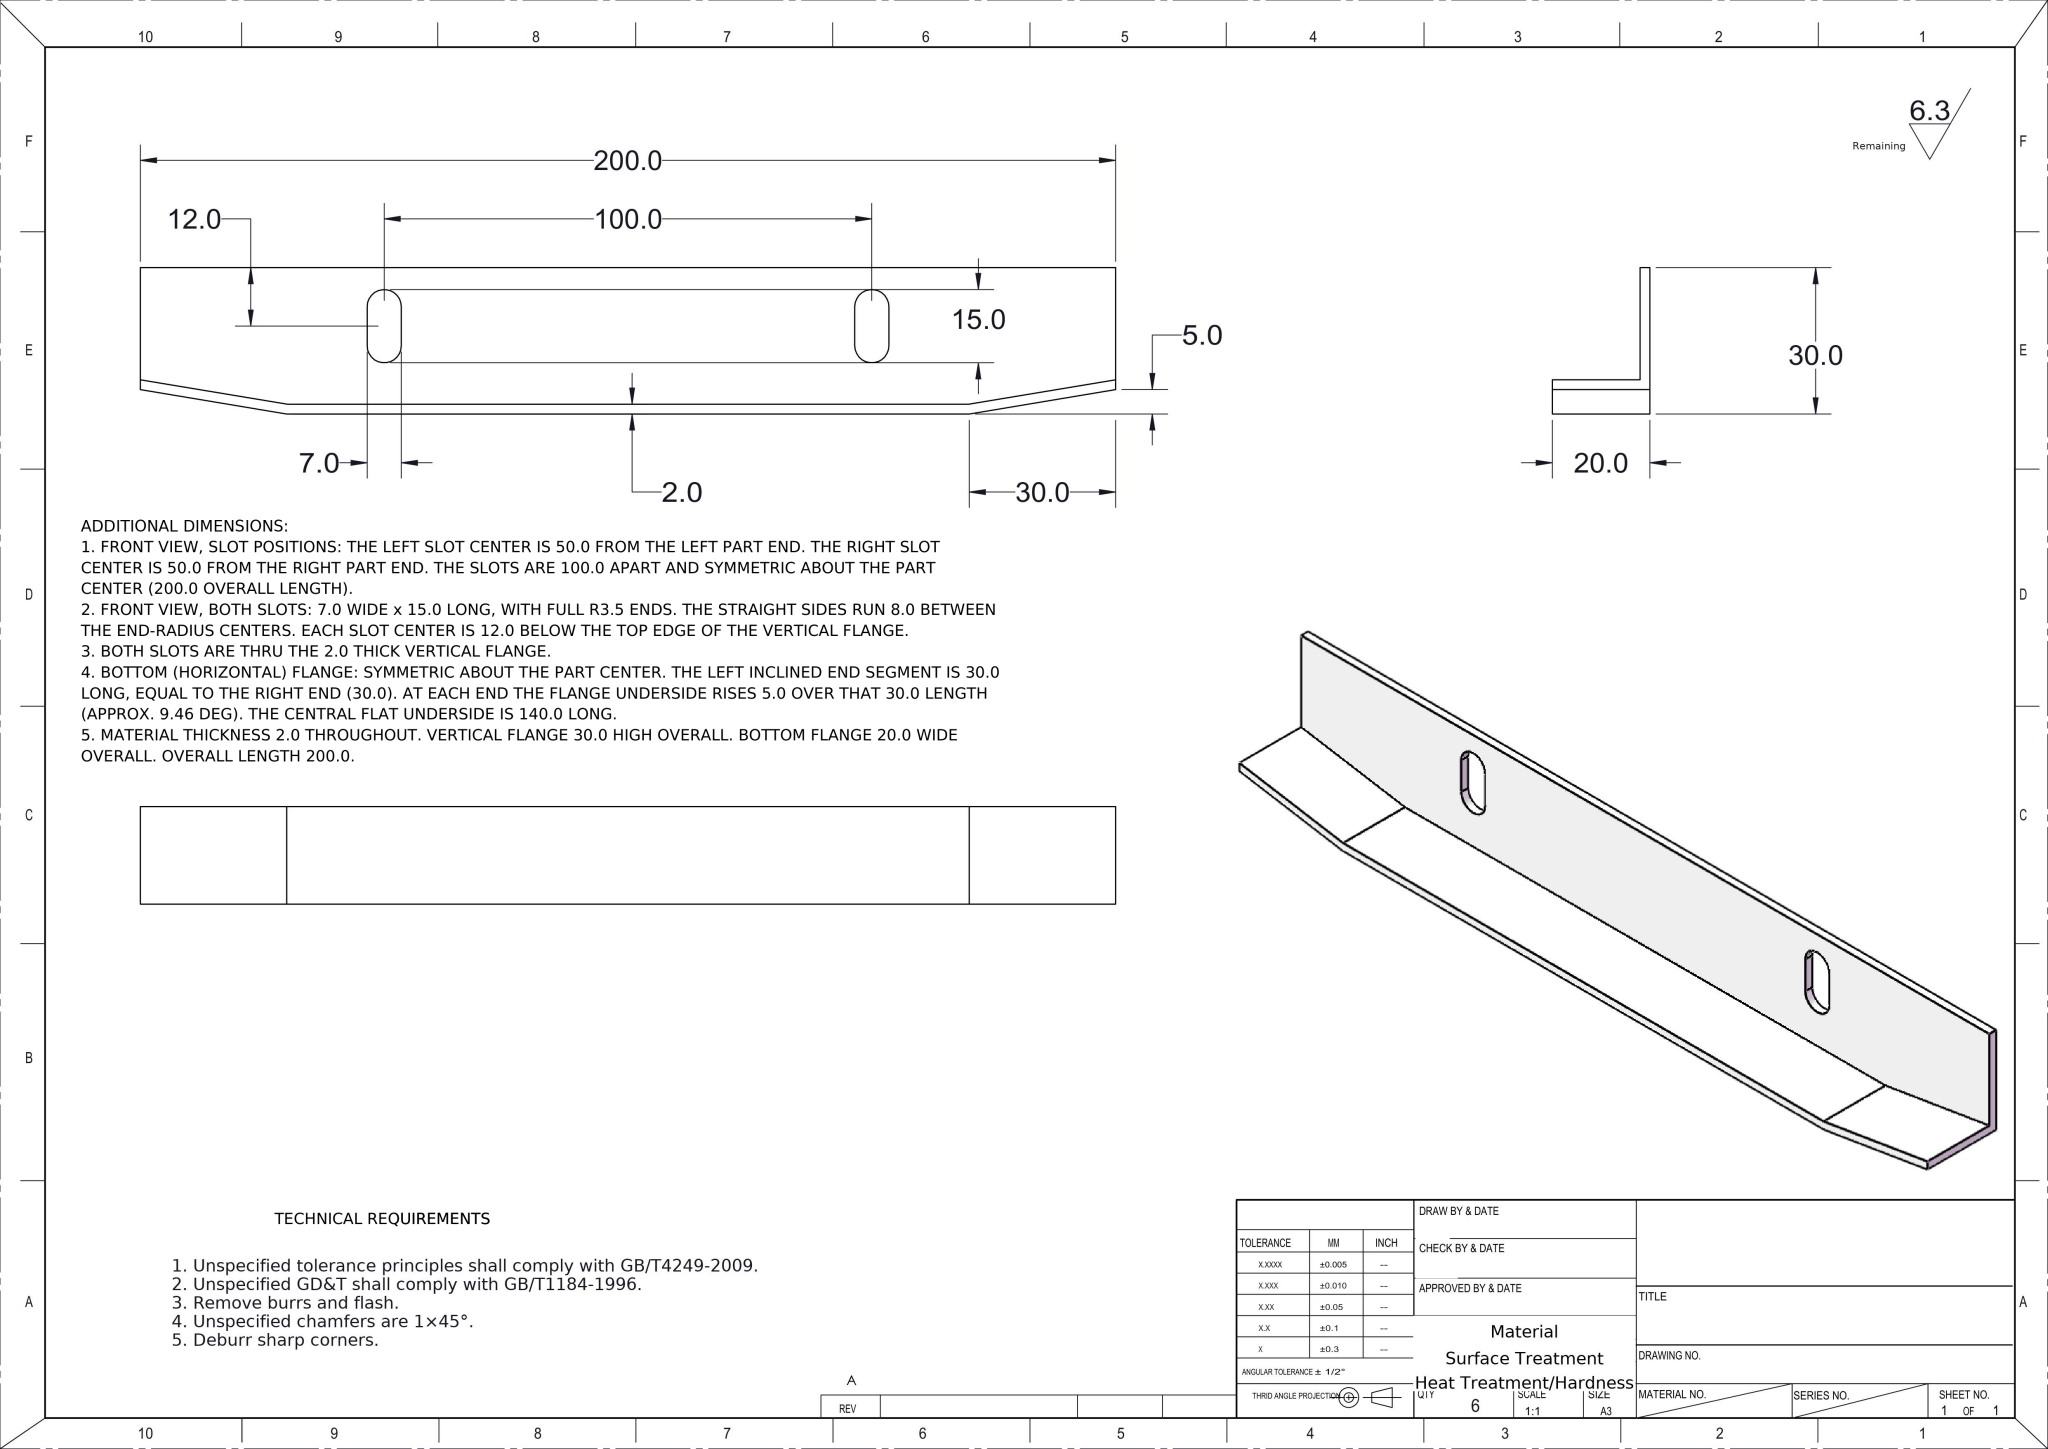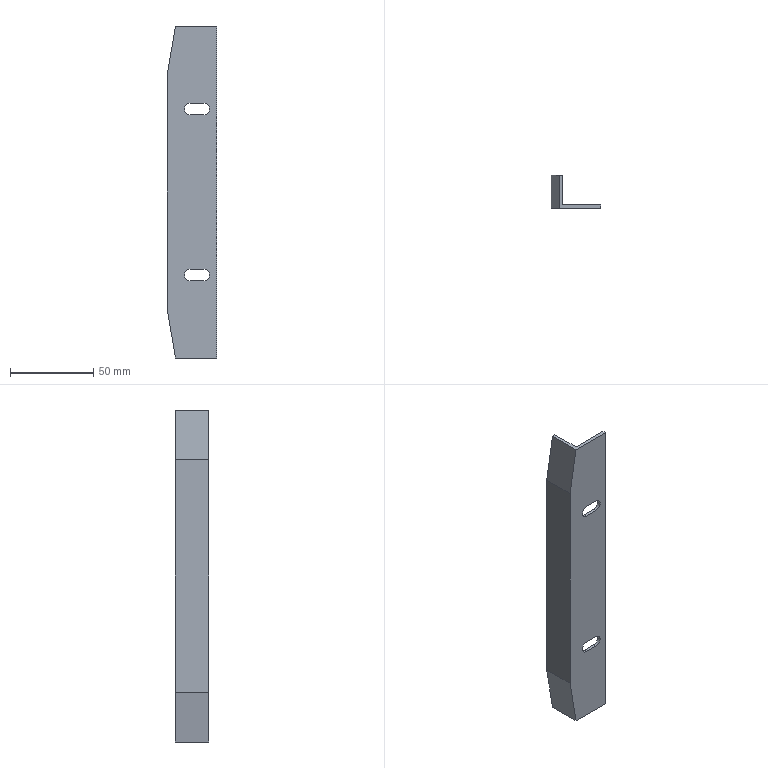Part | NX | mm | Angled Top Mounting Bracket | 1 solid | 20 faces | box 30 x 20 x 200 mm | volume 18552 mm3 | plane 16 | cylinder 4 | commonest cylinder face diameters 7 x4
STEP:
#1=COLOUR_RGB('',1.,1.,1.);
#2=FILL_AREA_STYLE_COLOUR('',#1);
#3=FILL_AREA_STYLE('',(#2));
#4=SURFACE_STYLE_FILL_AREA(#3);
#5=SURFACE_SIDE_STYLE('',(#4));
#6=SURFACE_STYLE_USAGE(.BOTH.,#5);
#7=PRESENTATION_STYLE_ASSIGNMENT((#6));
#8=CARTESIAN_POINT('',(7.028,20.,-100.));
#9=VERTEX_POINT('',#8);
#10=CARTESIAN_POINT('',(2.,20.,-69.834));
#11=VERTEX_POINT('',#10);
#12=CARTESIAN_POINT('',(1.973,20.,-69.671));
#13=DIRECTION('',(-0.1644,0.,0.9864));
#14=VECTOR('',#13,1000.);
#15=LINE('',#12,#14);
#16=EDGE_CURVE('',#9,#11,#15,.T.);
#17=ORIENTED_EDGE('',*,*,#16,.F.);
#18=CARTESIAN_POINT('',(5.,20.,-100.));
#19=VERTEX_POINT('',#18);
#20=CARTESIAN_POINT('',(0.,20.,-100.));
#21=DIRECTION('',(-1.,0.,0.));
#22=VECTOR('',#21,1000.);
#23=LINE('',#20,#22);
#24=EDGE_CURVE('',#9,#19,#23,.T.);
#25=ORIENTED_EDGE('',*,*,#24,.T.);
#26=CARTESIAN_POINT('',(0.,20.,-70.));
#27=VERTEX_POINT('',#26);
#28=CARTESIAN_POINT('',(0.,20.,-70.));
#29=DIRECTION('',(-0.1644,0.,0.9864));
#30=VECTOR('',#29,1000.);
#31=LINE('',#28,#30);
#32=EDGE_CURVE('',#19,#27,#31,.T.);
#33=ORIENTED_EDGE('',*,*,#32,.T.);
#34=CARTESIAN_POINT('',(0.,20.,70.));
#35=VERTEX_POINT('',#34);
#36=CARTESIAN_POINT('',(0.,20.,100.));
#37=DIRECTION('',(0.,0.,-1.));
#38=VECTOR('',#37,1000.);
#39=LINE('',#36,#38);
#40=EDGE_CURVE('',#35,#27,#39,.T.);
#41=ORIENTED_EDGE('',*,*,#40,.F.);
#42=CARTESIAN_POINT('',(5.,20.,100.));
#43=VERTEX_POINT('',#42);
#44=CARTESIAN_POINT('',(0.,20.,70.));
#45=DIRECTION('',(-0.1644,0.,-0.9864));
#46=VECTOR('',#45,1000.);
#47=LINE('',#44,#46);
#48=EDGE_CURVE('',#43,#35,#47,.T.);
#49=ORIENTED_EDGE('',*,*,#48,.F.);
#50=CARTESIAN_POINT('',(7.028,20.,100.));
#51=VERTEX_POINT('',#50);
#52=CARTESIAN_POINT('',(0.,20.,100.));
#53=DIRECTION('',(-1.,0.,0.));
#54=VECTOR('',#53,1000.);
#55=LINE('',#52,#54);
#56=EDGE_CURVE('',#51,#43,#55,.T.);
#57=ORIENTED_EDGE('',*,*,#56,.F.);
#58=CARTESIAN_POINT('',(2.,20.,69.834));
#59=VERTEX_POINT('',#58);
#60=CARTESIAN_POINT('',(1.973,20.,69.671));
#61=DIRECTION('',(-0.1644,0.,-0.9864));
#62=VECTOR('',#61,1000.);
#63=LINE('',#60,#62);
#64=EDGE_CURVE('',#51,#59,#63,.T.);
#65=ORIENTED_EDGE('',*,*,#64,.T.);
#66=CARTESIAN_POINT('',(2.,20.,100.));
#67=DIRECTION('',(0.,0.,-1.));
#68=VECTOR('',#67,1000.);
#69=LINE('',#66,#68);
#70=EDGE_CURVE('',#59,#11,#69,.T.);
#71=ORIENTED_EDGE('',*,*,#70,.T.);
#72=EDGE_LOOP('',(#17,#25,#33,#41,#49,#57,#65,#71));
#73=FACE_OUTER_BOUND('',#72,.T.);
#74=CARTESIAN_POINT('',(0.,20.,100.));
#75=DIRECTION('',(0.,-1.,0.));
#76=DIRECTION('',(0.,0.,-1.));
#77=AXIS2_PLACEMENT_3D('',#74,#75,#76);
#78=PLANE('',#77);
#79=ADVANCED_FACE('',(#73),#78,.F.);
#80=CARTESIAN_POINT('',(7.028,2.,-100.));
#81=VERTEX_POINT('',#80);
#82=CARTESIAN_POINT('',(7.028,0.,-100.));
#83=DIRECTION('',(0.,1.,0.));
#84=VECTOR('',#83,1000.);
#85=LINE('',#82,#84);
#86=EDGE_CURVE('',#81,#9,#85,.T.);
#87=ORIENTED_EDGE('',*,*,#86,.F.);
#88=CARTESIAN_POINT('',(30.,2.,-100.));
#89=VERTEX_POINT('',#88);
#90=CARTESIAN_POINT('',(0.,2.,-100.));
#91=DIRECTION('',(1.,0.,0.));
#92=VECTOR('',#91,1000.);
#93=LINE('',#90,#92);
#94=EDGE_CURVE('',#81,#89,#93,.T.);
#95=ORIENTED_EDGE('',*,*,#94,.T.);
#96=CARTESIAN_POINT('',(30.,0.,-100.));
#97=VERTEX_POINT('',#96);
#98=CARTESIAN_POINT('',(30.,20.,-100.));
#99=DIRECTION('',(-0.,1.,0.));
#100=VECTOR('',#99,1000.);
#101=LINE('',#98,#100);
#102=EDGE_CURVE('',#97,#89,#101,.T.);
#103=ORIENTED_EDGE('',*,*,#102,.F.);
#104=CARTESIAN_POINT('',(5.,0.,-100.));
#105=VERTEX_POINT('',#104);
#106=CARTESIAN_POINT('',(0.,0.,-100.));
#107=DIRECTION('',(1.,0.,0.));
#108=VECTOR('',#107,1000.);
#109=LINE('',#106,#108);
#110=EDGE_CURVE('',#105,#97,#109,.T.);
#111=ORIENTED_EDGE('',*,*,#110,.F.);
#112=CARTESIAN_POINT('',(5.,0.,-100.));
#113=DIRECTION('',(0.,1.,0.));
#114=VECTOR('',#113,1000.);
#115=LINE('',#112,#114);
#116=EDGE_CURVE('',#105,#19,#115,.T.);
#117=ORIENTED_EDGE('',*,*,#116,.T.);
#118=ORIENTED_EDGE('',*,*,#24,.F.);
#119=EDGE_LOOP('',(#87,#95,#103,#111,#117,#118));
#120=FACE_OUTER_BOUND('',#119,.T.);
#121=CARTESIAN_POINT('',(0.,0.,-100.));
#122=DIRECTION('',(0.,0.,-1.));
#123=DIRECTION('',(-1.,0.,0.));
#124=AXIS2_PLACEMENT_3D('',#121,#122,#123);
#125=PLANE('',#124);
#126=ADVANCED_FACE('',(#120),#125,.T.);
#127=CARTESIAN_POINT('',(30.,2.,100.));
#128=VERTEX_POINT('',#127);
#129=CARTESIAN_POINT('',(30.,2.,100.));
#130=DIRECTION('',(0.,0.,-1.));
#131=VECTOR('',#130,1000.);
#132=LINE('',#129,#131);
#133=EDGE_CURVE('',#128,#89,#132,.T.);
#134=ORIENTED_EDGE('',*,*,#133,.F.);
#135=CARTESIAN_POINT('',(30.,0.,100.));
#136=VERTEX_POINT('',#135);
#137=CARTESIAN_POINT('',(30.,20.,100.));
#138=DIRECTION('',(-0.,1.,0.));
#139=VECTOR('',#138,1000.);
#140=LINE('',#137,#139);
#141=EDGE_CURVE('',#136,#128,#140,.T.);
#142=ORIENTED_EDGE('',*,*,#141,.F.);
#143=CARTESIAN_POINT('',(30.,0.,100.));
#144=DIRECTION('',(0.,0.,-1.));
#145=VECTOR('',#144,1000.);
#146=LINE('',#143,#145);
#147=EDGE_CURVE('',#136,#97,#146,.T.);
#148=ORIENTED_EDGE('',*,*,#147,.T.);
#149=ORIENTED_EDGE('',*,*,#102,.T.);
#150=EDGE_LOOP('',(#134,#142,#148,#149));
#151=FACE_OUTER_BOUND('',#150,.T.);
#152=CARTESIAN_POINT('',(30.,20.,100.));
#153=DIRECTION('',(-1.,-0.,0.));
#154=DIRECTION('',(0.,-1.,0.));
#155=AXIS2_PLACEMENT_3D('',#152,#153,#154);
#156=PLANE('',#155);
#157=ADVANCED_FACE('',(#151),#156,.F.);
#158=CARTESIAN_POINT('',(0.,0.,-70.));
#159=VERTEX_POINT('',#158);
#160=CARTESIAN_POINT('',(0.,0.,-70.));
#161=DIRECTION('',(0.,1.,0.));
#162=VECTOR('',#161,1000.);
#163=LINE('',#160,#162);
#164=EDGE_CURVE('',#159,#27,#163,.T.);
#165=ORIENTED_EDGE('',*,*,#164,.F.);
#166=CARTESIAN_POINT('',(0.,0.,70.));
#167=VERTEX_POINT('',#166);
#168=CARTESIAN_POINT('',(0.,0.,100.));
#169=DIRECTION('',(0.,0.,-1.));
#170=VECTOR('',#169,1000.);
#171=LINE('',#168,#170);
#172=EDGE_CURVE('',#167,#159,#171,.T.);
#173=ORIENTED_EDGE('',*,*,#172,.F.);
#174=CARTESIAN_POINT('',(0.,0.,70.));
#175=DIRECTION('',(0.,1.,0.));
#176=VECTOR('',#175,1000.);
#177=LINE('',#174,#176);
#178=EDGE_CURVE('',#167,#35,#177,.T.);
#179=ORIENTED_EDGE('',*,*,#178,.T.);
#180=ORIENTED_EDGE('',*,*,#40,.T.);
#181=EDGE_LOOP('',(#165,#173,#179,#180));
#182=FACE_OUTER_BOUND('',#181,.T.);
#183=CARTESIAN_POINT('',(0.,20.,100.));
#184=DIRECTION('',(1.,0.,0.));
#185=DIRECTION('',(0.,0.,-1.));
#186=AXIS2_PLACEMENT_3D('',#183,#184,#185);
#187=PLANE('',#186);
#188=ADVANCED_FACE('',(#182),#187,.F.);
#189=CARTESIAN_POINT('',(22.,0.,-46.5));
#190=VERTEX_POINT('',#189);
#191=CARTESIAN_POINT('',(14.,0.,-46.5));
#192=VERTEX_POINT('',#191);
#193=CARTESIAN_POINT('',(22.,0.,-46.5));
#194=DIRECTION('',(-1.,0.,0.));
#195=VECTOR('',#194,1000.);
#196=LINE('',#193,#195);
#197=EDGE_CURVE('',#190,#192,#196,.T.);
#198=ORIENTED_EDGE('',*,*,#197,.F.);
#199=CARTESIAN_POINT('',(22.,0.,-53.5));
#200=VERTEX_POINT('',#199);
#201=CARTESIAN_POINT('',(22.,0.,-50.));
#202=DIRECTION('',(0.,-1.,0.));
#203=DIRECTION('',(0.,0.,1.));
#204=AXIS2_PLACEMENT_3D('',#201,#202,#203);
#205=CIRCLE('',#204,3.5);
#206=EDGE_CURVE('',#200,#190,#205,.T.);
#207=ORIENTED_EDGE('',*,*,#206,.F.);
#208=CARTESIAN_POINT('',(14.,0.,-53.5));
#209=VERTEX_POINT('',#208);
#210=CARTESIAN_POINT('',(22.,0.,-53.5));
#211=DIRECTION('',(1.,0.,0.));
#212=VECTOR('',#211,1000.);
#213=LINE('',#210,#212);
#214=EDGE_CURVE('',#209,#200,#213,.T.);
#215=ORIENTED_EDGE('',*,*,#214,.F.);
#216=CARTESIAN_POINT('',(14.,0.,-50.));
#217=DIRECTION('',(0.,-1.,0.));
#218=DIRECTION('',(0.,0.,1.));
#219=AXIS2_PLACEMENT_3D('',#216,#217,#218);
#220=CIRCLE('',#219,3.5);
#221=EDGE_CURVE('',#192,#209,#220,.T.);
#222=ORIENTED_EDGE('',*,*,#221,.F.);
#223=EDGE_LOOP('',(#198,#207,#215,#222));
#224=FACE_BOUND('',#223,.T.);
#225=CARTESIAN_POINT('',(22.,0.,53.5));
#226=VERTEX_POINT('',#225);
#227=CARTESIAN_POINT('',(14.,0.,53.5));
#228=VERTEX_POINT('',#227);
#229=CARTESIAN_POINT('',(22.,0.,53.5));
#230=DIRECTION('',(-1.,0.,0.));
#231=VECTOR('',#230,1000.);
#232=LINE('',#229,#231);
#233=EDGE_CURVE('',#226,#228,#232,.T.);
#234=ORIENTED_EDGE('',*,*,#233,.F.);
#235=CARTESIAN_POINT('',(22.,0.,46.5));
#236=VERTEX_POINT('',#235);
#237=CARTESIAN_POINT('',(22.,0.,50.));
#238=DIRECTION('',(0.,-1.,0.));
#239=DIRECTION('',(0.,0.,-1.));
#240=AXIS2_PLACEMENT_3D('',#237,#238,#239);
#241=CIRCLE('',#240,3.5);
#242=EDGE_CURVE('',#236,#226,#241,.T.);
#243=ORIENTED_EDGE('',*,*,#242,.F.);
#244=CARTESIAN_POINT('',(14.,0.,46.5));
#245=VERTEX_POINT('',#244);
#246=CARTESIAN_POINT('',(22.,0.,46.5));
#247=DIRECTION('',(1.,0.,0.));
#248=VECTOR('',#247,1000.);
#249=LINE('',#246,#248);
#250=EDGE_CURVE('',#245,#236,#249,.T.);
#251=ORIENTED_EDGE('',*,*,#250,.F.);
#252=CARTESIAN_POINT('',(14.,0.,50.));
#253=DIRECTION('',(0.,-1.,0.));
#254=DIRECTION('',(0.,0.,-1.));
#255=AXIS2_PLACEMENT_3D('',#252,#253,#254);
#256=CIRCLE('',#255,3.5);
#257=EDGE_CURVE('',#228,#245,#256,.T.);
#258=ORIENTED_EDGE('',*,*,#257,.F.);
#259=EDGE_LOOP('',(#234,#243,#251,#258));
#260=FACE_BOUND('',#259,.T.);
#261=CARTESIAN_POINT('',(0.,0.,-70.));
#262=DIRECTION('',(-0.1644,0.,0.9864));
#263=VECTOR('',#262,1000.);
#264=LINE('',#261,#263);
#265=EDGE_CURVE('',#105,#159,#264,.T.);
#266=ORIENTED_EDGE('',*,*,#265,.F.);
#267=ORIENTED_EDGE('',*,*,#110,.T.);
#268=ORIENTED_EDGE('',*,*,#147,.F.);
#269=CARTESIAN_POINT('',(5.,0.,100.));
#270=VERTEX_POINT('',#269);
#271=CARTESIAN_POINT('',(0.,0.,100.));
#272=DIRECTION('',(1.,0.,0.));
#273=VECTOR('',#272,1000.);
#274=LINE('',#271,#273);
#275=EDGE_CURVE('',#270,#136,#274,.T.);
#276=ORIENTED_EDGE('',*,*,#275,.F.);
#277=CARTESIAN_POINT('',(0.,0.,70.));
#278=DIRECTION('',(-0.1644,0.,-0.9864));
#279=VECTOR('',#278,1000.);
#280=LINE('',#277,#279);
#281=EDGE_CURVE('',#270,#167,#280,.T.);
#282=ORIENTED_EDGE('',*,*,#281,.T.);
#283=ORIENTED_EDGE('',*,*,#172,.T.);
#284=EDGE_LOOP('',(#266,#267,#268,#276,#282,#283));
#285=FACE_OUTER_BOUND('',#284,.T.);
#286=CARTESIAN_POINT('',(0.,0.,100.));
#287=DIRECTION('',(0.,1.,0.));
#288=DIRECTION('',(0.,0.,1.));
#289=AXIS2_PLACEMENT_3D('',#286,#287,#288);
#290=PLANE('',#289);
#291=ADVANCED_FACE('',(#224,#260,#285),#290,.F.);
#292=CARTESIAN_POINT('',(7.028,2.,100.));
#293=VERTEX_POINT('',#292);
#294=CARTESIAN_POINT('',(0.,2.,100.));
#295=DIRECTION('',(1.,0.,0.));
#296=VECTOR('',#295,1000.);
#297=LINE('',#294,#296);
#298=EDGE_CURVE('',#293,#128,#297,.T.);
#299=ORIENTED_EDGE('',*,*,#298,.F.);
#300=CARTESIAN_POINT('',(7.028,0.,100.));
#301=DIRECTION('',(0.,1.,0.));
#302=VECTOR('',#301,1000.);
#303=LINE('',#300,#302);
#304=EDGE_CURVE('',#293,#51,#303,.T.);
#305=ORIENTED_EDGE('',*,*,#304,.T.);
#306=ORIENTED_EDGE('',*,*,#56,.T.);
#307=CARTESIAN_POINT('',(5.,0.,100.));
#308=DIRECTION('',(0.,1.,0.));
#309=VECTOR('',#308,1000.);
#310=LINE('',#307,#309);
#311=EDGE_CURVE('',#270,#43,#310,.T.);
#312=ORIENTED_EDGE('',*,*,#311,.F.);
#313=ORIENTED_EDGE('',*,*,#275,.T.);
#314=ORIENTED_EDGE('',*,*,#141,.T.);
#315=EDGE_LOOP('',(#299,#305,#306,#312,#313,#314));
#316=FACE_OUTER_BOUND('',#315,.T.);
#317=CARTESIAN_POINT('',(0.,0.,100.));
#318=DIRECTION('',(0.,0.,-1.));
#319=DIRECTION('',(-1.,0.,0.));
#320=AXIS2_PLACEMENT_3D('',#317,#318,#319);
#321=PLANE('',#320);
#322=ADVANCED_FACE('',(#316),#321,.F.);
#323=ORIENTED_EDGE('',*,*,#48,.T.);
#324=ORIENTED_EDGE('',*,*,#178,.F.);
#325=ORIENTED_EDGE('',*,*,#281,.F.);
#326=ORIENTED_EDGE('',*,*,#311,.T.);
#327=EDGE_LOOP('',(#323,#324,#325,#326));
#328=FACE_OUTER_BOUND('',#327,.T.);
#329=CARTESIAN_POINT('',(0.,0.,70.));
#330=DIRECTION('',(0.9864,0.,-0.1644));
#331=DIRECTION('',(-0.1644,0.,-0.9864));
#332=AXIS2_PLACEMENT_3D('',#329,#330,#331);
#333=PLANE('',#332);
#334=ADVANCED_FACE('',(#328),#333,.F.);
#335=ORIENTED_EDGE('',*,*,#32,.F.);
#336=ORIENTED_EDGE('',*,*,#116,.F.);
#337=ORIENTED_EDGE('',*,*,#265,.T.);
#338=ORIENTED_EDGE('',*,*,#164,.T.);
#339=EDGE_LOOP('',(#335,#336,#337,#338));
#340=FACE_OUTER_BOUND('',#339,.T.);
#341=CARTESIAN_POINT('',(0.,0.,-70.));
#342=DIRECTION('',(-0.9864,0.,-0.1644));
#343=DIRECTION('',(-0.1644,0.,0.9864));
#344=AXIS2_PLACEMENT_3D('',#341,#342,#343);
#345=PLANE('',#344);
#346=ADVANCED_FACE('',(#340),#345,.T.);
#347=CARTESIAN_POINT('',(2.,2.,-69.834));
#348=VERTEX_POINT('',#347);
#349=CARTESIAN_POINT('',(2.,20.,-69.834));
#350=DIRECTION('',(0.,1.,0.));
#351=VECTOR('',#350,1000.);
#352=LINE('',#349,#351);
#353=EDGE_CURVE('',#348,#11,#352,.T.);
#354=ORIENTED_EDGE('',*,*,#353,.T.);
#355=ORIENTED_EDGE('',*,*,#70,.F.);
#356=CARTESIAN_POINT('',(2.,2.,69.834));
#357=VERTEX_POINT('',#356);
#358=CARTESIAN_POINT('',(2.,20.,69.834));
#359=DIRECTION('',(0.,1.,0.));
#360=VECTOR('',#359,1000.);
#361=LINE('',#358,#360);
#362=EDGE_CURVE('',#357,#59,#361,.T.);
#363=ORIENTED_EDGE('',*,*,#362,.F.);
#364=CARTESIAN_POINT('',(2.,2.,100.));
#365=DIRECTION('',(0.,0.,-1.));
#366=VECTOR('',#365,1000.);
#367=LINE('',#364,#366);
#368=EDGE_CURVE('',#357,#348,#367,.T.);
#369=ORIENTED_EDGE('',*,*,#368,.T.);
#370=EDGE_LOOP('',(#354,#355,#363,#369));
#371=FACE_OUTER_BOUND('',#370,.T.);
#372=CARTESIAN_POINT('',(2.,20.,100.));
#373=DIRECTION('',(1.,0.,0.));
#374=DIRECTION('',(0.,0.,-1.));
#375=AXIS2_PLACEMENT_3D('',#372,#373,#374);
#376=PLANE('',#375);
#377=ADVANCED_FACE('',(#371),#376,.T.);
#378=CARTESIAN_POINT('',(22.,2.,-53.5));
#379=VERTEX_POINT('',#378);
#380=CARTESIAN_POINT('',(22.,2.,-46.5));
#381=VERTEX_POINT('',#380);
#382=CARTESIAN_POINT('',(22.,2.,-50.));
#383=DIRECTION('',(0.,-1.,0.));
#384=DIRECTION('',(0.,0.,1.));
#385=AXIS2_PLACEMENT_3D('',#382,#383,#384);
#386=CIRCLE('',#385,3.5);
#387=EDGE_CURVE('',#379,#381,#386,.T.);
#388=ORIENTED_EDGE('',*,*,#387,.T.);
#389=CARTESIAN_POINT('',(14.,2.,-46.5));
#390=VERTEX_POINT('',#389);
#391=CARTESIAN_POINT('',(22.,2.,-46.5));
#392=DIRECTION('',(-1.,0.,0.));
#393=VECTOR('',#392,1000.);
#394=LINE('',#391,#393);
#395=EDGE_CURVE('',#381,#390,#394,.T.);
#396=ORIENTED_EDGE('',*,*,#395,.T.);
#397=CARTESIAN_POINT('',(14.,2.,-53.5));
#398=VERTEX_POINT('',#397);
#399=CARTESIAN_POINT('',(14.,2.,-50.));
#400=DIRECTION('',(0.,-1.,0.));
#401=DIRECTION('',(0.,0.,1.));
#402=AXIS2_PLACEMENT_3D('',#399,#400,#401);
#403=CIRCLE('',#402,3.5);
#404=EDGE_CURVE('',#390,#398,#403,.T.);
#405=ORIENTED_EDGE('',*,*,#404,.T.);
#406=CARTESIAN_POINT('',(22.,2.,-53.5));
#407=DIRECTION('',(1.,0.,0.));
#408=VECTOR('',#407,1000.);
#409=LINE('',#406,#408);
#410=EDGE_CURVE('',#398,#379,#409,.T.);
#411=ORIENTED_EDGE('',*,*,#410,.T.);
#412=EDGE_LOOP('',(#388,#396,#405,#411));
#413=FACE_BOUND('',#412,.T.);
#414=CARTESIAN_POINT('',(22.,2.,46.5));
#415=VERTEX_POINT('',#414);
#416=CARTESIAN_POINT('',(22.,2.,53.5));
#417=VERTEX_POINT('',#416);
#418=CARTESIAN_POINT('',(22.,2.,50.));
#419=DIRECTION('',(0.,-1.,0.));
#420=DIRECTION('',(-0.,0.,1.));
#421=AXIS2_PLACEMENT_3D('',#418,#419,#420);
#422=CIRCLE('',#421,3.5);
#423=EDGE_CURVE('',#415,#417,#422,.T.);
#424=ORIENTED_EDGE('',*,*,#423,.T.);
#425=CARTESIAN_POINT('',(14.,2.,53.5));
#426=VERTEX_POINT('',#425);
#427=CARTESIAN_POINT('',(22.,2.,53.5));
#428=DIRECTION('',(-1.,0.,0.));
#429=VECTOR('',#428,1000.);
#430=LINE('',#427,#429);
#431=EDGE_CURVE('',#417,#426,#430,.T.);
#432=ORIENTED_EDGE('',*,*,#431,.T.);
#433=CARTESIAN_POINT('',(14.,2.,46.5));
#434=VERTEX_POINT('',#433);
#435=CARTESIAN_POINT('',(14.,2.,50.));
#436=DIRECTION('',(0.,-1.,0.));
#437=DIRECTION('',(0.,0.,1.));
#438=AXIS2_PLACEMENT_3D('',#435,#436,#437);
#439=CIRCLE('',#438,3.5);
#440=EDGE_CURVE('',#426,#434,#439,.T.);
#441=ORIENTED_EDGE('',*,*,#440,.T.);
#442=CARTESIAN_POINT('',(22.,2.,46.5));
#443=DIRECTION('',(1.,0.,0.));
#444=VECTOR('',#443,1000.);
#445=LINE('',#442,#444);
#446=EDGE_CURVE('',#434,#415,#445,.T.);
#447=ORIENTED_EDGE('',*,*,#446,.T.);
#448=EDGE_LOOP('',(#424,#432,#441,#447));
#449=FACE_BOUND('',#448,.T.);
#450=CARTESIAN_POINT('',(-25.595,2.,95.734));
#451=DIRECTION('',(-0.1644,0.,0.9864));
#452=VECTOR('',#451,1000.);
#453=LINE('',#450,#452);
#454=EDGE_CURVE('',#81,#348,#453,.T.);
#455=ORIENTED_EDGE('',*,*,#454,.T.);
#456=ORIENTED_EDGE('',*,*,#368,.F.);
#457=CARTESIAN_POINT('',(6.838,2.,98.86));
#458=DIRECTION('',(-0.1644,0.,-0.9864));
#459=VECTOR('',#458,1000.);
#460=LINE('',#457,#459);
#461=EDGE_CURVE('',#293,#357,#460,.T.);
#462=ORIENTED_EDGE('',*,*,#461,.F.);
#463=ORIENTED_EDGE('',*,*,#298,.T.);
#464=ORIENTED_EDGE('',*,*,#133,.T.);
#465=ORIENTED_EDGE('',*,*,#94,.F.);
#466=EDGE_LOOP('',(#455,#456,#462,#463,#464,#465));
#467=FACE_OUTER_BOUND('',#466,.T.);
#468=CARTESIAN_POINT('',(0.,2.,100.));
#469=DIRECTION('',(0.,1.,0.));
#470=DIRECTION('',(0.,0.,1.));
#471=AXIS2_PLACEMENT_3D('',#468,#469,#470);
#472=PLANE('',#471);
#473=ADVANCED_FACE('',(#413,#449,#467),#472,.T.);
#474=ORIENTED_EDGE('',*,*,#64,.F.);
#475=ORIENTED_EDGE('',*,*,#304,.F.);
#476=ORIENTED_EDGE('',*,*,#461,.T.);
#477=ORIENTED_EDGE('',*,*,#362,.T.);
#478=EDGE_LOOP('',(#474,#475,#476,#477));
#479=FACE_OUTER_BOUND('',#478,.T.);
#480=CARTESIAN_POINT('',(1.973,0.,69.671));
#481=DIRECTION('',(0.9864,0.,-0.1644));
#482=DIRECTION('',(-0.1644,0.,-0.9864));
#483=AXIS2_PLACEMENT_3D('',#480,#481,#482);
#484=PLANE('',#483);
#485=ADVANCED_FACE('',(#479),#484,.T.);
#486=ORIENTED_EDGE('',*,*,#16,.T.);
#487=ORIENTED_EDGE('',*,*,#353,.F.);
#488=ORIENTED_EDGE('',*,*,#454,.F.);
#489=ORIENTED_EDGE('',*,*,#86,.T.);
#490=EDGE_LOOP('',(#486,#487,#488,#489));
#491=FACE_OUTER_BOUND('',#490,.T.);
#492=CARTESIAN_POINT('',(1.973,0.,-69.671));
#493=DIRECTION('',(-0.9864,0.,-0.1644));
#494=DIRECTION('',(-0.1644,0.,0.9864));
#495=AXIS2_PLACEMENT_3D('',#492,#493,#494);
#496=PLANE('',#495);
#497=ADVANCED_FACE('',(#491),#496,.F.);
#498=CARTESIAN_POINT('',(22.,20.001,46.5));
#499=DIRECTION('',(0.,-1.,0.));
#500=VECTOR('',#499,1000.);
#501=LINE('',#498,#500);
#502=EDGE_CURVE('',#415,#236,#501,.T.);
#503=ORIENTED_EDGE('',*,*,#502,.T.);
#504=ORIENTED_EDGE('',*,*,#242,.T.);
#505=CARTESIAN_POINT('',(22.,20.001,53.5));
#506=DIRECTION('',(0.,-1.,0.));
#507=VECTOR('',#506,1000.);
#508=LINE('',#505,#507);
#509=EDGE_CURVE('',#417,#226,#508,.T.);
#510=ORIENTED_EDGE('',*,*,#509,.F.);
#511=ORIENTED_EDGE('',*,*,#423,.F.);
#512=EDGE_LOOP('',(#503,#504,#510,#511));
#513=FACE_OUTER_BOUND('',#512,.T.);
#514=CARTESIAN_POINT('',(22.,20.001,50.));
#515=DIRECTION('',(0.,-1.,0.));
#516=DIRECTION('',(0.,0.,-1.));
#517=AXIS2_PLACEMENT_3D('',#514,#515,#516);
#518=CYLINDRICAL_SURFACE('',#517,3.5);
#519=ADVANCED_FACE('',(#513),#518,.F.);
#520=CARTESIAN_POINT('',(14.,20.001,46.5));
#521=DIRECTION('',(0.,-1.,0.));
#522=VECTOR('',#521,1000.);
#523=LINE('',#520,#522);
#524=EDGE_CURVE('',#434,#245,#523,.T.);
#525=ORIENTED_EDGE('',*,*,#524,.T.);
#526=ORIENTED_EDGE('',*,*,#250,.T.);
#527=ORIENTED_EDGE('',*,*,#502,.F.);
#528=ORIENTED_EDGE('',*,*,#446,.F.);
#529=EDGE_LOOP('',(#525,#526,#527,#528));
#530=FACE_OUTER_BOUND('',#529,.T.);
#531=CARTESIAN_POINT('',(22.,20.001,46.5));
#532=DIRECTION('',(0.,0.,-1.));
#533=DIRECTION('',(-1.,0.,0.));
#534=AXIS2_PLACEMENT_3D('',#531,#532,#533);
#535=PLANE('',#534);
#536=ADVANCED_FACE('',(#530),#535,.F.);
#537=CARTESIAN_POINT('',(14.,20.001,53.5));
#538=DIRECTION('',(0.,-1.,0.));
#539=VECTOR('',#538,1000.);
#540=LINE('',#537,#539);
#541=EDGE_CURVE('',#426,#228,#540,.T.);
#542=ORIENTED_EDGE('',*,*,#541,.T.);
#543=ORIENTED_EDGE('',*,*,#257,.T.);
#544=ORIENTED_EDGE('',*,*,#524,.F.);
#545=ORIENTED_EDGE('',*,*,#440,.F.);
#546=EDGE_LOOP('',(#542,#543,#544,#545));
#547=FACE_OUTER_BOUND('',#546,.T.);
#548=CARTESIAN_POINT('',(14.,20.001,50.));
#549=DIRECTION('',(0.,-1.,0.));
#550=DIRECTION('',(0.,0.,-1.));
#551=AXIS2_PLACEMENT_3D('',#548,#549,#550);
#552=CYLINDRICAL_SURFACE('',#551,3.5);
#553=ADVANCED_FACE('',(#547),#552,.F.);
#554=ORIENTED_EDGE('',*,*,#509,.T.);
#555=ORIENTED_EDGE('',*,*,#233,.T.);
#556=ORIENTED_EDGE('',*,*,#541,.F.);
#557=ORIENTED_EDGE('',*,*,#431,.F.);
#558=EDGE_LOOP('',(#554,#555,#556,#557));
#559=FACE_OUTER_BOUND('',#558,.T.);
#560=CARTESIAN_POINT('',(22.,20.001,53.5));
#561=DIRECTION('',(0.,0.,1.));
#562=DIRECTION('',(1.,0.,0.));
#563=AXIS2_PLACEMENT_3D('',#560,#561,#562);
#564=PLANE('',#563);
#565=ADVANCED_FACE('',(#559),#564,.F.);
#566=CARTESIAN_POINT('',(22.,20.001,-53.5));
#567=DIRECTION('',(0.,-1.,0.));
#568=VECTOR('',#567,1000.);
#569=LINE('',#566,#568);
#570=EDGE_CURVE('',#379,#200,#569,.T.);
#571=ORIENTED_EDGE('',*,*,#570,.T.);
#572=ORIENTED_EDGE('',*,*,#206,.T.);
#573=CARTESIAN_POINT('',(22.,20.001,-46.5));
#574=DIRECTION('',(0.,-1.,0.));
#575=VECTOR('',#574,1000.);
#576=LINE('',#573,#575);
#577=EDGE_CURVE('',#381,#190,#576,.T.);
#578=ORIENTED_EDGE('',*,*,#577,.F.);
#579=ORIENTED_EDGE('',*,*,#387,.F.);
#580=EDGE_LOOP('',(#571,#572,#578,#579));
#581=FACE_OUTER_BOUND('',#580,.T.);
#582=CARTESIAN_POINT('',(22.,20.001,-50.));
#583=DIRECTION('',(0.,-1.,0.));
#584=DIRECTION('',(0.,0.,-1.));
#585=AXIS2_PLACEMENT_3D('',#582,#583,#584);
#586=CYLINDRICAL_SURFACE('',#585,3.5);
#587=ADVANCED_FACE('',(#581),#586,.F.);
#588=CARTESIAN_POINT('',(14.,20.001,-53.5));
#589=DIRECTION('',(0.,-1.,0.));
#590=VECTOR('',#589,1000.);
#591=LINE('',#588,#590);
#592=EDGE_CURVE('',#398,#209,#591,.T.);
#593=ORIENTED_EDGE('',*,*,#592,.T.);
#594=ORIENTED_EDGE('',*,*,#214,.T.);
#595=ORIENTED_EDGE('',*,*,#570,.F.);
#596=ORIENTED_EDGE('',*,*,#410,.F.);
#597=EDGE_LOOP('',(#593,#594,#595,#596));
#598=FACE_OUTER_BOUND('',#597,.T.);
#599=CARTESIAN_POINT('',(22.,20.001,-53.5));
#600=DIRECTION('',(0.,0.,-1.));
#601=DIRECTION('',(-1.,0.,0.));
#602=AXIS2_PLACEMENT_3D('',#599,#600,#601);
#603=PLANE('',#602);
#604=ADVANCED_FACE('',(#598),#603,.F.);
#605=CARTESIAN_POINT('',(14.,20.001,-46.5));
#606=DIRECTION('',(0.,-1.,0.));
#607=VECTOR('',#606,1000.);
#608=LINE('',#605,#607);
#609=EDGE_CURVE('',#390,#192,#608,.T.);
#610=ORIENTED_EDGE('',*,*,#609,.T.);
#611=ORIENTED_EDGE('',*,*,#221,.T.);
#612=ORIENTED_EDGE('',*,*,#592,.F.);
#613=ORIENTED_EDGE('',*,*,#404,.F.);
#614=EDGE_LOOP('',(#610,#611,#612,#613));
#615=FACE_OUTER_BOUND('',#614,.T.);
#616=CARTESIAN_POINT('',(14.,20.001,-50.));
#617=DIRECTION('',(0.,-1.,0.));
#618=DIRECTION('',(0.,0.,-1.));
#619=AXIS2_PLACEMENT_3D('',#616,#617,#618);
#620=CYLINDRICAL_SURFACE('',#619,3.5);
#621=ADVANCED_FACE('',(#615),#620,.F.);
#622=ORIENTED_EDGE('',*,*,#577,.T.);
#623=ORIENTED_EDGE('',*,*,#197,.T.);
#624=ORIENTED_EDGE('',*,*,#609,.F.);
#625=ORIENTED_EDGE('',*,*,#395,.F.);
#626=EDGE_LOOP('',(#622,#623,#624,#625));
#627=FACE_OUTER_BOUND('',#626,.T.);
#628=CARTESIAN_POINT('',(22.,20.001,-46.5));
#629=DIRECTION('',(0.,0.,1.));
#630=DIRECTION('',(1.,0.,0.));
#631=AXIS2_PLACEMENT_3D('',#628,#629,#630);
#632=PLANE('',#631);
#633=ADVANCED_FACE('',(#627),#632,.F.);
#634=CLOSED_SHELL('',(#79,#126,#157,#188,#291,#322,#334,#346,#377,#473,#485,#497,#519,#536,#553,#565,#587,#604,#621,#633));
#635=MANIFOLD_SOLID_BREP('',#634);
#636=STYLED_ITEM('',(#7),#635);
#637=PRESENTATION_LAYER_ASSIGNMENT('','',(#636));
#638=(LENGTH_UNIT()NAMED_UNIT(*)SI_UNIT(.MILLI.,.METRE.));
#639=UNCERTAINTY_MEASURE_WITH_UNIT(LENGTH_MEASURE(0.00001),#638,'','');
#640=(NAMED_UNIT(*)PLANE_ANGLE_UNIT()SI_UNIT($,.RADIAN.));
#641=(NAMED_UNIT(*)SI_UNIT($,.STERADIAN.)SOLID_ANGLE_UNIT());
#642=(GEOMETRIC_REPRESENTATION_CONTEXT(3)GLOBAL_UNCERTAINTY_ASSIGNED_CONTEXT((#639))GLOBAL_UNIT_ASSIGNED_CONTEXT((#638,#640,#641))REPRESENTATION_CONTEXT('',''));
#643=MECHANICAL_DESIGN_GEOMETRIC_PRESENTATION_REPRESENTATION('',(#636),#642);
#644=COLOUR_RGB('',1.,1.,1.);
#645=FILL_AREA_STYLE_COLOUR('',#644);
#646=FILL_AREA_STYLE('',(#645));
#647=SURFACE_STYLE_FILL_AREA(#646);
#648=SURFACE_SIDE_STYLE('',(#647));
#649=SURFACE_STYLE_USAGE(.BOTH.,#648);
#650=PRESENTATION_STYLE_ASSIGNMENT((#649));
#651=CARTESIAN_POINT('',(0.,0.,0.));
#652=DIRECTION('',(0.,0.,1.));
#653=DIRECTION('',(1.,0.,0.));
#654=AXIS2_PLACEMENT_3D('',#651,#652,#653);
#655=(LENGTH_UNIT()NAMED_UNIT(*)SI_UNIT(.MILLI.,.METRE.));
#656=UNCERTAINTY_MEASURE_WITH_UNIT(LENGTH_MEASURE(0.00001),#655,'','');
#657=(NAMED_UNIT(*)PLANE_ANGLE_UNIT()SI_UNIT($,.RADIAN.));
#658=(NAMED_UNIT(*)SI_UNIT($,.STERADIAN.)SOLID_ANGLE_UNIT());
#659=(GEOMETRIC_REPRESENTATION_CONTEXT(3)GLOBAL_UNCERTAINTY_ASSIGNED_CONTEXT((#656))GLOBAL_UNIT_ASSIGNED_CONTEXT((#655,#657,#658))REPRESENTATION_CONTEXT('',''));
#660=ADVANCED_BREP_SHAPE_REPRESENTATION('',(#635,#654),#659);
#661=STYLED_ITEM('',(#650),#660);
#662=(LENGTH_UNIT()NAMED_UNIT(*)SI_UNIT(.MILLI.,.METRE.));
#663=UNCERTAINTY_MEASURE_WITH_UNIT(LENGTH_MEASURE(0.00001),#662,'','');
#664=(NAMED_UNIT(*)PLANE_ANGLE_UNIT()SI_UNIT($,.RADIAN.));
#665=(NAMED_UNIT(*)SI_UNIT($,.STERADIAN.)SOLID_ANGLE_UNIT());
#666=(GEOMETRIC_REPRESENTATION_CONTEXT(3)GLOBAL_UNCERTAINTY_ASSIGNED_CONTEXT((#663))GLOBAL_UNIT_ASSIGNED_CONTEXT((#662,#664,#665))REPRESENTATION_CONTEXT('',''));
#667=MECHANICAL_DESIGN_GEOMETRIC_PRESENTATION_REPRESENTATION('',(#661),#666);
#668=PRESENTATION_LAYER_ASSIGNMENT('','',(#661));